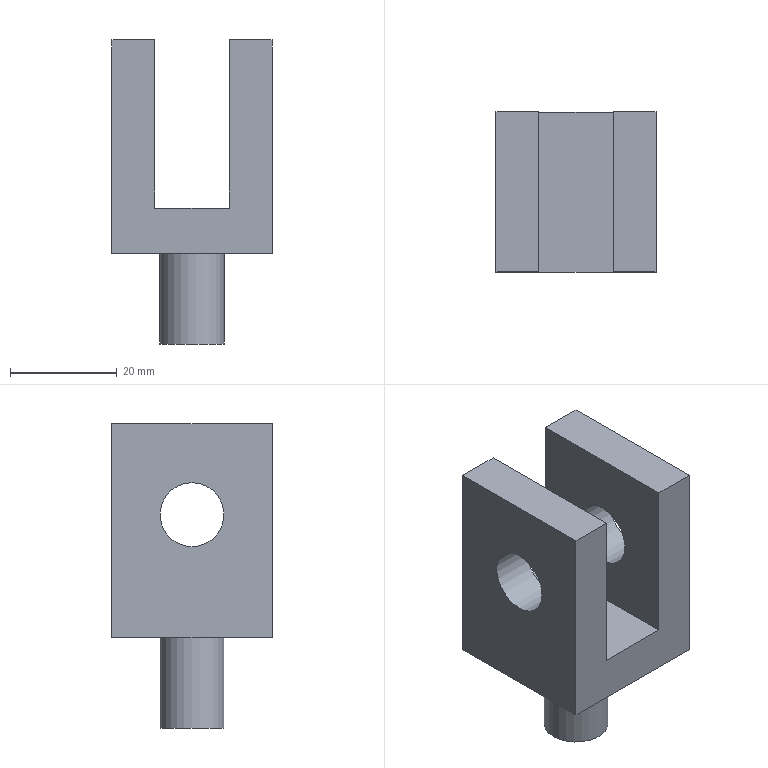Component | NX | HINGE_LINK | 1 solid | 14 faces | box 30 x 30 x 57 mm | volume 22883 mm3 | plane 11 | cylinder 3 | commonest cylinder face diameters 12 x3
STEP:
#1=CARTESIAN_POINT('',(0.,0.,0.));
#2=DIRECTION('',(0.,0.,1.));
#3=DIRECTION('',(1.,0.,0.));
#4=AXIS2_PLACEMENT_3D('',#1,#2,#3);
#5=CARTESIAN_POINT('',(545.625,-110.909,-15.057));
#6=VERTEX_POINT('',#5);
#7=CARTESIAN_POINT('',(553.625,-110.909,-15.057));
#8=VERTEX_POINT('',#7);
#9=CARTESIAN_POINT('',(545.625,-110.909,-15.057));
#10=DIRECTION('',(1.,0.,0.));
#11=VECTOR('',#10,1.);
#12=LINE('',#9,#11);
#13=CARTESIAN_POINT('',(560.625,-95.909,-15.057));
#14=DIRECTION('',(0.,0.,1.));
#15=DIRECTION('',(1.,0.,0.));
#16=AXIS2_PLACEMENT_3D('',#13,#14,#15);
#17=PLANE('',#16);
#18=CARTESIAN_POINT('',(-15.,-15.));
#19=DIRECTION('',(1.,0.));
#20=VECTOR('',#19,1.);
#21=LINE('',#18,#20);
#22=(GEOMETRIC_REPRESENTATION_CONTEXT(2)PARAMETRIC_REPRESENTATION_CONTEXT()REPRESENTATION_CONTEXT('',''));
#23=DEFINITIONAL_REPRESENTATION('',(#21),#22);
#24=PCURVE('',#17,#23);
#25=CARTESIAN_POINT('',(545.625,-110.909,-10.057));
#26=DIRECTION('',(0.,1.,0.));
#27=DIRECTION('',(0.,0.,1.));
#28=AXIS2_PLACEMENT_3D('',#25,#26,#27);
#29=PLANE('',#28);
#30=CARTESIAN_POINT('',(-5.,0.));
#31=DIRECTION('',(0.,1.));
#32=VECTOR('',#31,1.);
#33=LINE('',#30,#32);
#34=(GEOMETRIC_REPRESENTATION_CONTEXT(2)PARAMETRIC_REPRESENTATION_CONTEXT()REPRESENTATION_CONTEXT('',''));
#35=DEFINITIONAL_REPRESENTATION('',(#33),#34);
#36=PCURVE('',#29,#35);
#37=SURFACE_CURVE('',#12,(#24,#36),.PCURVE_S1.);
#38=EDGE_CURVE('',#6,#8,#37,.T.);
#39=ORIENTED_EDGE('',*,*,#38,.T.);
#40=CARTESIAN_POINT('',(553.625,-80.909,-15.057));
#41=VERTEX_POINT('',#40);
#42=CARTESIAN_POINT('',(553.625,-95.909,-15.057));
#43=DIRECTION('',(0.,1.,0.));
#44=VECTOR('',#43,1.);
#45=LINE('',#42,#44);
#46=CARTESIAN_POINT('',(-7.,0.));
#47=DIRECTION('',(0.,1.));
#48=VECTOR('',#47,1.);
#49=LINE('',#46,#48);
#50=(GEOMETRIC_REPRESENTATION_CONTEXT(2)PARAMETRIC_REPRESENTATION_CONTEXT()REPRESENTATION_CONTEXT('',''));
#51=DEFINITIONAL_REPRESENTATION('',(#49),#50);
#52=PCURVE('',#17,#51);
#53=CARTESIAN_POINT('',(553.625,-95.909,-72.057));
#54=DIRECTION('',(1.,0.,0.));
#55=DIRECTION('',(0.,0.,-1.));
#56=AXIS2_PLACEMENT_3D('',#53,#54,#55);
#57=PLANE('',#56);
#58=CARTESIAN_POINT('',(-57.,0.));
#59=DIRECTION('',(0.,1.));
#60=VECTOR('',#59,1.);
#61=LINE('',#58,#60);
#62=(GEOMETRIC_REPRESENTATION_CONTEXT(2)PARAMETRIC_REPRESENTATION_CONTEXT()REPRESENTATION_CONTEXT('',''));
#63=DEFINITIONAL_REPRESENTATION('',(#61),#62);
#64=PCURVE('',#57,#63);
#65=SURFACE_CURVE('',#45,(#52,#64),.PCURVE_S1.);
#66=EDGE_CURVE('',#8,#41,#65,.T.);
#67=ORIENTED_EDGE('',*,*,#66,.T.);
#68=CARTESIAN_POINT('',(545.625,-80.909,-15.057));
#69=VERTEX_POINT('',#68);
#70=CARTESIAN_POINT('',(575.625,-80.909,-15.057));
#71=DIRECTION('',(-1.,0.,0.));
#72=VECTOR('',#71,1.);
#73=LINE('',#70,#72);
#74=CARTESIAN_POINT('',(15.,15.));
#75=DIRECTION('',(-1.,0.));
#76=VECTOR('',#75,1.);
#77=LINE('',#74,#76);
#78=(GEOMETRIC_REPRESENTATION_CONTEXT(2)PARAMETRIC_REPRESENTATION_CONTEXT()REPRESENTATION_CONTEXT('',''));
#79=DEFINITIONAL_REPRESENTATION('',(#77),#78);
#80=PCURVE('',#17,#79);
#81=CARTESIAN_POINT('',(575.625,-80.909,-10.057));
#82=DIRECTION('',(0.,-1.,0.));
#83=DIRECTION('',(0.,0.,-1.));
#84=AXIS2_PLACEMENT_3D('',#81,#82,#83);
#85=PLANE('',#84);
#86=CARTESIAN_POINT('',(5.,0.));
#87=DIRECTION('',(0.,-1.));
#88=VECTOR('',#87,1.);
#89=LINE('',#86,#88);
#90=(GEOMETRIC_REPRESENTATION_CONTEXT(2)PARAMETRIC_REPRESENTATION_CONTEXT()REPRESENTATION_CONTEXT('',''));
#91=DEFINITIONAL_REPRESENTATION('',(#89),#90);
#92=PCURVE('',#85,#91);
#93=SURFACE_CURVE('',#73,(#80,#92),.PCURVE_S1.);
#94=EDGE_CURVE('',#41,#69,#93,.T.);
#95=ORIENTED_EDGE('',*,*,#94,.T.);
#96=CARTESIAN_POINT('',(545.625,-80.909,-15.057));
#97=DIRECTION('',(0.,-1.,0.));
#98=VECTOR('',#97,1.);
#99=LINE('',#96,#98);
#100=CARTESIAN_POINT('',(-15.,15.));
#101=DIRECTION('',(0.,-1.));
#102=VECTOR('',#101,1.);
#103=LINE('',#100,#102);
#104=(GEOMETRIC_REPRESENTATION_CONTEXT(2)PARAMETRIC_REPRESENTATION_CONTEXT()REPRESENTATION_CONTEXT('',''));
#105=DEFINITIONAL_REPRESENTATION('',(#103),#104);
#106=PCURVE('',#17,#105);
#107=CARTESIAN_POINT('',(545.625,-80.909,-10.057));
#108=DIRECTION('',(1.,0.,0.));
#109=DIRECTION('',(0.,0.,-1.));
#110=AXIS2_PLACEMENT_3D('',#107,#108,#109);
#111=PLANE('',#110);
#112=CARTESIAN_POINT('',(5.,0.));
#113=DIRECTION('',(0.,-1.));
#114=VECTOR('',#113,1.);
#115=LINE('',#112,#114);
#116=(GEOMETRIC_REPRESENTATION_CONTEXT(2)PARAMETRIC_REPRESENTATION_CONTEXT()REPRESENTATION_CONTEXT('',''));
#117=DEFINITIONAL_REPRESENTATION('',(#115),#116);
#118=PCURVE('',#111,#117);
#119=SURFACE_CURVE('',#99,(#106,#118),.PCURVE_S1.);
#120=EDGE_CURVE('',#69,#6,#119,.T.);
#121=ORIENTED_EDGE('',*,*,#120,.T.);
#122=EDGE_LOOP('',(#39,#67,#95,#121));
#123=FACE_BOUND('',#122,.T.);
#124=ADVANCED_FACE('',(#123),#17,.T.);
#125=CARTESIAN_POINT('',(566.625,-95.909,-72.057));
#126=VERTEX_POINT('',#125);
#127=CARTESIAN_POINT('',(560.625,-95.909,-72.057));
#128=DIRECTION('',(0.,0.,1.));
#129=DIRECTION('',(1.,0.,0.));
#130=AXIS2_PLACEMENT_3D('',#127,#128,#129);
#131=CIRCLE('',#130,6.);
#132=CARTESIAN_POINT('',(560.625,-95.909,-72.057));
#133=DIRECTION('',(0.,0.,-1.));
#134=DIRECTION('',(-1.,0.,0.));
#135=AXIS2_PLACEMENT_3D('',#132,#133,#134);
#136=PLANE('',#135);
#137=CARTESIAN_POINT('',(-6.,0.));
#138=CARTESIAN_POINT('',(-6.,10.392));
#139=CARTESIAN_POINT('',(3.,5.196));
#140=CARTESIAN_POINT('',(12.,0.));
#141=CARTESIAN_POINT('',(3.,-5.196));
#142=CARTESIAN_POINT('',(-6.,-10.392));
#143=CARTESIAN_POINT('',(-6.,0.));
#144=(BOUNDED_CURVE()B_SPLINE_CURVE(2,(#137,#138,#139,#140,#141,#142,#143),.UNSPECIFIED.,.T.,.F.)B_SPLINE_CURVE_WITH_KNOTS((1,2,2,2,2,1),(-2.094,0.,2.094,4.189,6.283,8.378),.UNSPECIFIED.)CURVE()GEOMETRIC_REPRESENTATION_ITEM()RATIONAL_B_SPLINE_CURVE((1.,0.5,1.,0.5,1.,0.5,1.))REPRESENTATION_ITEM(''));
#145=(GEOMETRIC_REPRESENTATION_CONTEXT(2)PARAMETRIC_REPRESENTATION_CONTEXT()REPRESENTATION_CONTEXT('',''));
#146=DEFINITIONAL_REPRESENTATION('',(#144),#145);
#147=PCURVE('',#136,#146);
#148=CARTESIAN_POINT('',(560.625,-95.909,-72.057));
#149=DIRECTION('',(0.,0.,1.));
#150=DIRECTION('',(1.,0.,0.));
#151=AXIS2_PLACEMENT_3D('',#148,#149,#150);
#152=CYLINDRICAL_SURFACE('',#151,6.);
#153=CARTESIAN_POINT('',(0.,0.));
#154=DIRECTION('',(1.,0.));
#155=VECTOR('',#154,1.);
#156=LINE('',#153,#155);
#157=(GEOMETRIC_REPRESENTATION_CONTEXT(2)PARAMETRIC_REPRESENTATION_CONTEXT()REPRESENTATION_CONTEXT('',''));
#158=DEFINITIONAL_REPRESENTATION('',(#156),#157);
#159=PCURVE('',#152,#158);
#160=SURFACE_CURVE('',#131,(#147,#159),.PCURVE_S1.);
#161=EDGE_CURVE('',#126,#126,#160,.T.);
#162=ORIENTED_EDGE('',*,*,#161,.F.);
#163=EDGE_LOOP('',(#162));
#164=FACE_BOUND('',#163,.T.);
#165=ADVANCED_FACE('',(#164),#136,.T.);
#166=CARTESIAN_POINT('',(566.625,-95.909,-55.057));
#167=VERTEX_POINT('',#166);
#168=CARTESIAN_POINT('',(560.625,-95.909,-55.057));
#169=DIRECTION('',(0.,0.,-1.));
#170=DIRECTION('',(1.,0.,0.));
#171=AXIS2_PLACEMENT_3D('',#168,#169,#170);
#172=CIRCLE('',#171,6.);
#173=CARTESIAN_POINT('',(6.283,17.));
#174=DIRECTION('',(-1.,0.));
#175=VECTOR('',#174,1.);
#176=LINE('',#173,#175);
#177=(GEOMETRIC_REPRESENTATION_CONTEXT(2)PARAMETRIC_REPRESENTATION_CONTEXT()REPRESENTATION_CONTEXT('',''));
#178=DEFINITIONAL_REPRESENTATION('',(#176),#177);
#179=PCURVE('',#152,#178);
#180=CARTESIAN_POINT('',(560.625,-95.909,-55.057));
#181=DIRECTION('',(0.,0.,1.));
#182=DIRECTION('',(1.,0.,0.));
#183=AXIS2_PLACEMENT_3D('',#180,#181,#182);
#184=PLANE('',#183);
#185=CARTESIAN_POINT('',(6.,0.));
#186=CARTESIAN_POINT('',(6.,-10.392));
#187=CARTESIAN_POINT('',(-3.,-5.196));
#188=CARTESIAN_POINT('',(-12.,-0.));
#189=CARTESIAN_POINT('',(-3.,5.196));
#190=CARTESIAN_POINT('',(6.,10.392));
#191=CARTESIAN_POINT('',(6.,0.));
#192=(BOUNDED_CURVE()B_SPLINE_CURVE(2,(#185,#186,#187,#188,#189,#190,#191),.UNSPECIFIED.,.T.,.F.)B_SPLINE_CURVE_WITH_KNOTS((1,2,2,2,2,1),(-2.094,0.,2.094,4.189,6.283,8.378),.UNSPECIFIED.)CURVE()GEOMETRIC_REPRESENTATION_ITEM()RATIONAL_B_SPLINE_CURVE((1.,0.5,1.,0.5,1.,0.5,1.))REPRESENTATION_ITEM(''));
#193=(GEOMETRIC_REPRESENTATION_CONTEXT(2)PARAMETRIC_REPRESENTATION_CONTEXT()REPRESENTATION_CONTEXT('',''));
#194=DEFINITIONAL_REPRESENTATION('',(#192),#193);
#195=PCURVE('',#184,#194);
#196=SURFACE_CURVE('',#172,(#179,#195),.PCURVE_S1.);
#197=EDGE_CURVE('',#167,#167,#196,.T.);
#198=ORIENTED_EDGE('',*,*,#197,.T.);
#199=CARTESIAN_POINT('',(566.625,-95.909,-72.057));
#200=CARTESIAN_POINT('',(566.625,-95.909,-55.057));
#201=B_SPLINE_CURVE_WITH_KNOTS('',1,(#199,#200),.UNSPECIFIED.,.F.,.F.,(2,2),(0.,17.),.PIECEWISE_BEZIER_KNOTS.);
#202=CARTESIAN_POINT('',(0.,0.));
#203=DIRECTION('',(0.,1.));
#204=VECTOR('',#203,1.);
#205=LINE('',#202,#204);
#206=(GEOMETRIC_REPRESENTATION_CONTEXT(2)PARAMETRIC_REPRESENTATION_CONTEXT()REPRESENTATION_CONTEXT('',''));
#207=DEFINITIONAL_REPRESENTATION('',(#205),#206);
#208=PCURVE('',#152,#207);
#209=CARTESIAN_POINT('',(6.283,0.));
#210=DIRECTION('',(0.,1.));
#211=VECTOR('',#210,1.);
#212=LINE('',#209,#211);
#213=(GEOMETRIC_REPRESENTATION_CONTEXT(2)PARAMETRIC_REPRESENTATION_CONTEXT()REPRESENTATION_CONTEXT('',''));
#214=DEFINITIONAL_REPRESENTATION('',(#212),#213);
#215=PCURVE('',#152,#214);
#216=SEAM_CURVE('',#201,(#208,#215),.PCURVE_S1.);
#217=EDGE_CURVE('',#126,#167,#216,.T.);
#218=ORIENTED_EDGE('',*,*,#217,.F.);
#219=ORIENTED_EDGE('',*,*,#161,.T.);
#220=ORIENTED_EDGE('',*,*,#217,.T.);
#221=EDGE_LOOP('',(#198,#218,#219,#220));
#222=FACE_BOUND('',#221,.T.);
#223=ADVANCED_FACE('',(#222),#152,.T.);
#224=CARTESIAN_POINT('',(545.625,-95.909,-38.057));
#225=VERTEX_POINT('',#224);
#226=CARTESIAN_POINT('',(545.625,-95.909,-32.057));
#227=DIRECTION('',(-1.,0.,0.));
#228=DIRECTION('',(0.,0.,-1.));
#229=AXIS2_PLACEMENT_3D('',#226,#227,#228);
#230=CIRCLE('',#229,6.);
#231=CARTESIAN_POINT('',(28.,-15.));
#232=CARTESIAN_POINT('',(28.,-25.392));
#233=CARTESIAN_POINT('',(19.,-20.196));
#234=CARTESIAN_POINT('',(10.,-15.));
#235=CARTESIAN_POINT('',(19.,-9.804));
#236=CARTESIAN_POINT('',(28.,-4.608));
#237=CARTESIAN_POINT('',(28.,-15.));
#238=(BOUNDED_CURVE()B_SPLINE_CURVE(2,(#231,#232,#233,#234,#235,#236,#237),.UNSPECIFIED.,.T.,.F.)B_SPLINE_CURVE_WITH_KNOTS((1,2,2,2,2,1),(-2.094,0.,2.094,4.189,6.283,8.378),.UNSPECIFIED.)CURVE()GEOMETRIC_REPRESENTATION_ITEM()RATIONAL_B_SPLINE_CURVE((1.,0.5,1.,0.5,1.,0.5,1.))REPRESENTATION_ITEM(''));
#239=(GEOMETRIC_REPRESENTATION_CONTEXT(2)PARAMETRIC_REPRESENTATION_CONTEXT()REPRESENTATION_CONTEXT('',''));
#240=DEFINITIONAL_REPRESENTATION('',(#238),#239);
#241=PCURVE('',#111,#240);
#242=CARTESIAN_POINT('',(591.625,-95.909,-32.057));
#243=DIRECTION('',(-1.,0.,0.));
#244=DIRECTION('',(0.,0.,1.));
#245=AXIS2_PLACEMENT_3D('',#242,#243,#244);
#246=CYLINDRICAL_SURFACE('',#245,6.);
#247=CARTESIAN_POINT('',(3.142,46.));
#248=DIRECTION('',(1.,0.));
#249=VECTOR('',#248,1.);
#250=LINE('',#247,#249);
#251=(GEOMETRIC_REPRESENTATION_CONTEXT(2)PARAMETRIC_REPRESENTATION_CONTEXT()REPRESENTATION_CONTEXT('',''));
#252=DEFINITIONAL_REPRESENTATION('',(#250),#251);
#253=PCURVE('',#246,#252);
#254=SURFACE_CURVE('',#230,(#241,#253),.PCURVE_S1.);
#255=EDGE_CURVE('',#225,#225,#254,.T.);
#256=ORIENTED_EDGE('',*,*,#255,.F.);
#257=EDGE_LOOP('',(#256));
#258=FACE_BOUND('',#257,.T.);
#259=CARTESIAN_POINT('',(545.625,-80.909,-55.057));
#260=VERTEX_POINT('',#259);
#261=CARTESIAN_POINT('',(545.625,-110.909,-55.057));
#262=VERTEX_POINT('',#261);
#263=CARTESIAN_POINT('',(545.625,-80.909,-55.057));
#264=DIRECTION('',(0.,-1.,0.));
#265=VECTOR('',#264,1.);
#266=LINE('',#263,#265);
#267=CARTESIAN_POINT('',(45.,0.));
#268=DIRECTION('',(0.,-1.));
#269=VECTOR('',#268,1.);
#270=LINE('',#267,#269);
#271=(GEOMETRIC_REPRESENTATION_CONTEXT(2)PARAMETRIC_REPRESENTATION_CONTEXT()REPRESENTATION_CONTEXT('',''));
#272=DEFINITIONAL_REPRESENTATION('',(#270),#271);
#273=PCURVE('',#111,#272);
#274=CARTESIAN_POINT('',(-15.,15.));
#275=DIRECTION('',(0.,-1.));
#276=VECTOR('',#275,1.);
#277=LINE('',#274,#276);
#278=(GEOMETRIC_REPRESENTATION_CONTEXT(2)PARAMETRIC_REPRESENTATION_CONTEXT()REPRESENTATION_CONTEXT('',''));
#279=DEFINITIONAL_REPRESENTATION('',(#277),#278);
#280=PCURVE('',#184,#279);
#281=SURFACE_CURVE('',#266,(#273,#280),.PCURVE_S1.);
#282=EDGE_CURVE('',#260,#262,#281,.T.);
#283=ORIENTED_EDGE('',*,*,#282,.T.);
#284=CARTESIAN_POINT('',(545.625,-110.909,-10.057));
#285=DIRECTION('',(0.,0.,-1.));
#286=VECTOR('',#285,1.);
#287=LINE('',#284,#286);
#288=CARTESIAN_POINT('',(0.,-30.));
#289=DIRECTION('',(1.,0.));
#290=VECTOR('',#289,1.);
#291=LINE('',#288,#290);
#292=(GEOMETRIC_REPRESENTATION_CONTEXT(2)PARAMETRIC_REPRESENTATION_CONTEXT()REPRESENTATION_CONTEXT('',''));
#293=DEFINITIONAL_REPRESENTATION('',(#291),#292);
#294=PCURVE('',#111,#293);
#295=CARTESIAN_POINT('',(0.,0.));
#296=DIRECTION('',(-1.,0.));
#297=VECTOR('',#296,1.);
#298=LINE('',#295,#297);
#299=(GEOMETRIC_REPRESENTATION_CONTEXT(2)PARAMETRIC_REPRESENTATION_CONTEXT()REPRESENTATION_CONTEXT('',''));
#300=DEFINITIONAL_REPRESENTATION('',(#298),#299);
#301=PCURVE('',#29,#300);
#302=SURFACE_CURVE('',#287,(#294,#301),.PCURVE_S1.);
#303=EDGE_CURVE('',#6,#262,#302,.T.);
#304=ORIENTED_EDGE('',*,*,#303,.F.);
#305=ORIENTED_EDGE('',*,*,#120,.F.);
#306=CARTESIAN_POINT('',(545.625,-80.909,-10.057));
#307=DIRECTION('',(0.,0.,-1.));
#308=VECTOR('',#307,1.);
#309=LINE('',#306,#308);
#310=CARTESIAN_POINT('',(0.,0.));
#311=DIRECTION('',(1.,0.));
#312=VECTOR('',#311,1.);
#313=LINE('',#310,#312);
#314=(GEOMETRIC_REPRESENTATION_CONTEXT(2)PARAMETRIC_REPRESENTATION_CONTEXT()REPRESENTATION_CONTEXT('',''));
#315=DEFINITIONAL_REPRESENTATION('',(#313),#314);
#316=PCURVE('',#111,#315);
#317=CARTESIAN_POINT('',(0.,-30.));
#318=DIRECTION('',(1.,0.));
#319=VECTOR('',#318,1.);
#320=LINE('',#317,#319);
#321=(GEOMETRIC_REPRESENTATION_CONTEXT(2)PARAMETRIC_REPRESENTATION_CONTEXT()REPRESENTATION_CONTEXT('',''));
#322=DEFINITIONAL_REPRESENTATION('',(#320),#321);
#323=PCURVE('',#85,#322);
#324=SURFACE_CURVE('',#309,(#316,#323),.PCURVE_S1.);
#325=EDGE_CURVE('',#69,#260,#324,.T.);
#326=ORIENTED_EDGE('',*,*,#325,.T.);
#327=EDGE_LOOP('',(#283,#304,#305,#326));
#328=FACE_BOUND('',#327,.T.);
#329=ADVANCED_FACE('',(#258,#328),#111,.F.);
#330=CARTESIAN_POINT('',(567.625,-110.909,-15.057));
#331=VERTEX_POINT('',#330);
#332=CARTESIAN_POINT('',(575.625,-110.909,-15.057));
#333=VERTEX_POINT('',#332);
#334=CARTESIAN_POINT('',(545.625,-110.909,-15.057));
#335=DIRECTION('',(1.,0.,0.));
#336=VECTOR('',#335,1.);
#337=LINE('',#334,#336);
#338=CARTESIAN_POINT('',(-5.,0.));
#339=DIRECTION('',(0.,1.));
#340=VECTOR('',#339,1.);
#341=LINE('',#338,#340);
#342=(GEOMETRIC_REPRESENTATION_CONTEXT(2)PARAMETRIC_REPRESENTATION_CONTEXT()REPRESENTATION_CONTEXT('',''));
#343=DEFINITIONAL_REPRESENTATION('',(#341),#342);
#344=PCURVE('',#29,#343);
#345=CARTESIAN_POINT('',(560.625,-95.909,-15.057));
#346=DIRECTION('',(0.,0.,1.));
#347=DIRECTION('',(1.,0.,0.));
#348=AXIS2_PLACEMENT_3D('',#345,#346,#347);
#349=PLANE('',#348);
#350=CARTESIAN_POINT('',(-15.,-15.));
#351=DIRECTION('',(1.,0.));
#352=VECTOR('',#351,1.);
#353=LINE('',#350,#352);
#354=(GEOMETRIC_REPRESENTATION_CONTEXT(2)PARAMETRIC_REPRESENTATION_CONTEXT()REPRESENTATION_CONTEXT('',''));
#355=DEFINITIONAL_REPRESENTATION('',(#353),#354);
#356=PCURVE('',#349,#355);
#357=SURFACE_CURVE('',#337,(#344,#356),.PCURVE_S1.);
#358=EDGE_CURVE('',#331,#333,#357,.T.);
#359=ORIENTED_EDGE('',*,*,#358,.F.);
#360=CARTESIAN_POINT('',(567.625,-110.909,-46.557));
#361=VERTEX_POINT('',#360);
#362=CARTESIAN_POINT('',(567.625,-110.909,-10.057));
#363=DIRECTION('',(0.,0.,-1.));
#364=VECTOR('',#363,1.);
#365=LINE('',#362,#364);
#366=CARTESIAN_POINT('',(0.,22.));
#367=DIRECTION('',(-1.,0.));
#368=VECTOR('',#367,1.);
#369=LINE('',#366,#368);
#370=(GEOMETRIC_REPRESENTATION_CONTEXT(2)PARAMETRIC_REPRESENTATION_CONTEXT()REPRESENTATION_CONTEXT('',''));
#371=DEFINITIONAL_REPRESENTATION('',(#369),#370);
#372=PCURVE('',#29,#371);
#373=CARTESIAN_POINT('',(567.625,-95.909,-72.057));
#374=DIRECTION('',(1.,0.,0.));
#375=DIRECTION('',(0.,0.,-1.));
#376=AXIS2_PLACEMENT_3D('',#373,#374,#375);
#377=PLANE('',#376);
#378=CARTESIAN_POINT('',(-62.,-15.));
#379=DIRECTION('',(1.,0.));
#380=VECTOR('',#379,1.);
#381=LINE('',#378,#380);
#382=(GEOMETRIC_REPRESENTATION_CONTEXT(2)PARAMETRIC_REPRESENTATION_CONTEXT()REPRESENTATION_CONTEXT('',''));
#383=DEFINITIONAL_REPRESENTATION('',(#381),#382);
#384=PCURVE('',#377,#383);
#385=SURFACE_CURVE('',#365,(#372,#384),.PCURVE_S1.);
#386=EDGE_CURVE('',#331,#361,#385,.T.);
#387=ORIENTED_EDGE('',*,*,#386,.T.);
#388=CARTESIAN_POINT('',(553.625,-110.909,-46.557));
#389=VERTEX_POINT('',#388);
#390=CARTESIAN_POINT('',(545.625,-110.909,-46.557));
#391=DIRECTION('',(1.,0.,0.));
#392=VECTOR('',#391,1.);
#393=LINE('',#390,#392);
#394=CARTESIAN_POINT('',(-36.5,0.));
#395=DIRECTION('',(0.,1.));
#396=VECTOR('',#395,1.);
#397=LINE('',#394,#396);
#398=(GEOMETRIC_REPRESENTATION_CONTEXT(2)PARAMETRIC_REPRESENTATION_CONTEXT()REPRESENTATION_CONTEXT('',''));
#399=DEFINITIONAL_REPRESENTATION('',(#397),#398);
#400=PCURVE('',#29,#399);
#401=CARTESIAN_POINT('',(567.625,-135.909,-46.557));
#402=DIRECTION('',(0.,-0.,1.));
#403=DIRECTION('',(0.,-1.,-0.));
#404=AXIS2_PLACEMENT_3D('',#401,#402,#403);
#405=PLANE('',#404);
#406=CARTESIAN_POINT('',(-25.,-22.));
#407=DIRECTION('',(0.,1.));
#408=VECTOR('',#407,1.);
#409=LINE('',#406,#408);
#410=(GEOMETRIC_REPRESENTATION_CONTEXT(2)PARAMETRIC_REPRESENTATION_CONTEXT()REPRESENTATION_CONTEXT('',''));
#411=DEFINITIONAL_REPRESENTATION('',(#409),#410);
#412=PCURVE('',#405,#411);
#413=SURFACE_CURVE('',#393,(#400,#412),.PCURVE_S1.);
#414=EDGE_CURVE('',#389,#361,#413,.T.);
#415=ORIENTED_EDGE('',*,*,#414,.F.);
#416=CARTESIAN_POINT('',(553.625,-110.909,-10.057));
#417=DIRECTION('',(0.,0.,-1.));
#418=VECTOR('',#417,1.);
#419=LINE('',#416,#418);
#420=CARTESIAN_POINT('',(0.,8.));
#421=DIRECTION('',(-1.,0.));
#422=VECTOR('',#421,1.);
#423=LINE('',#420,#422);
#424=(GEOMETRIC_REPRESENTATION_CONTEXT(2)PARAMETRIC_REPRESENTATION_CONTEXT()REPRESENTATION_CONTEXT('',''));
#425=DEFINITIONAL_REPRESENTATION('',(#423),#424);
#426=PCURVE('',#29,#425);
#427=CARTESIAN_POINT('',(-62.,-15.));
#428=DIRECTION('',(1.,0.));
#429=VECTOR('',#428,1.);
#430=LINE('',#427,#429);
#431=(GEOMETRIC_REPRESENTATION_CONTEXT(2)PARAMETRIC_REPRESENTATION_CONTEXT()REPRESENTATION_CONTEXT('',''));
#432=DEFINITIONAL_REPRESENTATION('',(#430),#431);
#433=PCURVE('',#57,#432);
#434=SURFACE_CURVE('',#419,(#426,#433),.PCURVE_S1.);
#435=EDGE_CURVE('',#8,#389,#434,.T.);
#436=ORIENTED_EDGE('',*,*,#435,.F.);
#437=ORIENTED_EDGE('',*,*,#38,.F.);
#438=ORIENTED_EDGE('',*,*,#303,.T.);
#439=CARTESIAN_POINT('',(575.625,-110.909,-55.057));
#440=VERTEX_POINT('',#439);
#441=CARTESIAN_POINT('',(545.625,-110.909,-55.057));
#442=DIRECTION('',(1.,0.,0.));
#443=VECTOR('',#442,1.);
#444=LINE('',#441,#443);
#445=CARTESIAN_POINT('',(-45.,0.));
#446=DIRECTION('',(0.,1.));
#447=VECTOR('',#446,1.);
#448=LINE('',#445,#447);
#449=(GEOMETRIC_REPRESENTATION_CONTEXT(2)PARAMETRIC_REPRESENTATION_CONTEXT()REPRESENTATION_CONTEXT('',''));
#450=DEFINITIONAL_REPRESENTATION('',(#448),#449);
#451=PCURVE('',#29,#450);
#452=CARTESIAN_POINT('',(-15.,-15.));
#453=DIRECTION('',(1.,0.));
#454=VECTOR('',#453,1.);
#455=LINE('',#452,#454);
#456=(GEOMETRIC_REPRESENTATION_CONTEXT(2)PARAMETRIC_REPRESENTATION_CONTEXT()REPRESENTATION_CONTEXT('',''));
#457=DEFINITIONAL_REPRESENTATION('',(#455),#456);
#458=PCURVE('',#184,#457);
#459=SURFACE_CURVE('',#444,(#451,#458),.PCURVE_S1.);
#460=EDGE_CURVE('',#262,#440,#459,.T.);
#461=ORIENTED_EDGE('',*,*,#460,.T.);
#462=CARTESIAN_POINT('',(575.625,-110.909,-10.057));
#463=DIRECTION('',(0.,0.,-1.));
#464=VECTOR('',#463,1.);
#465=LINE('',#462,#464);
#466=CARTESIAN_POINT('',(0.,30.));
#467=DIRECTION('',(-1.,0.));
#468=VECTOR('',#467,1.);
#469=LINE('',#466,#468);
#470=(GEOMETRIC_REPRESENTATION_CONTEXT(2)PARAMETRIC_REPRESENTATION_CONTEXT()REPRESENTATION_CONTEXT('',''));
#471=DEFINITIONAL_REPRESENTATION('',(#469),#470);
#472=PCURVE('',#29,#471);
#473=CARTESIAN_POINT('',(575.625,-110.909,-10.057));
#474=DIRECTION('',(-1.,0.,0.));
#475=DIRECTION('',(0.,0.,1.));
#476=AXIS2_PLACEMENT_3D('',#473,#474,#475);
#477=PLANE('',#476);
#478=CARTESIAN_POINT('',(0.,0.));
#479=DIRECTION('',(-1.,0.));
#480=VECTOR('',#479,1.);
#481=LINE('',#478,#480);
#482=(GEOMETRIC_REPRESENTATION_CONTEXT(2)PARAMETRIC_REPRESENTATION_CONTEXT()REPRESENTATION_CONTEXT('',''));
#483=DEFINITIONAL_REPRESENTATION('',(#481),#482);
#484=PCURVE('',#477,#483);
#485=SURFACE_CURVE('',#465,(#472,#484),.PCURVE_S1.);
#486=EDGE_CURVE('',#333,#440,#485,.T.);
#487=ORIENTED_EDGE('',*,*,#486,.F.);
#488=EDGE_LOOP('',(#359,#387,#415,#436,#437,#438,#461,#487));
#489=FACE_BOUND('',#488,.T.);
#490=ADVANCED_FACE('',(#489),#29,.F.);
#491=CARTESIAN_POINT('',(575.625,-95.909,-26.057));
#492=VERTEX_POINT('',#491);
#493=CARTESIAN_POINT('',(575.625,-95.909,-32.057));
#494=DIRECTION('',(1.,0.,0.));
#495=DIRECTION('',(0.,0.,1.));
#496=AXIS2_PLACEMENT_3D('',#493,#494,#495);
#497=CIRCLE('',#496,6.);
#498=CARTESIAN_POINT('',(-16.,15.));
#499=CARTESIAN_POINT('',(-16.,4.608));
#500=CARTESIAN_POINT('',(-25.,9.804));
#501=CARTESIAN_POINT('',(-34.,15.));
#502=CARTESIAN_POINT('',(-25.,20.196));
#503=CARTESIAN_POINT('',(-16.,25.392));
#504=CARTESIAN_POINT('',(-16.,15.));
#505=(BOUNDED_CURVE()B_SPLINE_CURVE(2,(#498,#499,#500,#501,#502,#503,#504),.UNSPECIFIED.,.T.,.F.)B_SPLINE_CURVE_WITH_KNOTS((1,2,2,2,2,1),(-2.094,0.,2.094,4.189,6.283,8.378),.UNSPECIFIED.)CURVE()GEOMETRIC_REPRESENTATION_ITEM()RATIONAL_B_SPLINE_CURVE((1.,0.5,1.,0.5,1.,0.5,1.))REPRESENTATION_ITEM(''));
#506=(GEOMETRIC_REPRESENTATION_CONTEXT(2)PARAMETRIC_REPRESENTATION_CONTEXT()REPRESENTATION_CONTEXT('',''));
#507=DEFINITIONAL_REPRESENTATION('',(#505),#506);
#508=PCURVE('',#477,#507);
#509=CARTESIAN_POINT('',(591.625,-95.909,-32.057));
#510=DIRECTION('',(-1.,0.,0.));
#511=DIRECTION('',(0.,0.,1.));
#512=AXIS2_PLACEMENT_3D('',#509,#510,#511);
#513=CYLINDRICAL_SURFACE('',#512,6.);
#514=CARTESIAN_POINT('',(6.283,16.));
#515=DIRECTION('',(-1.,0.));
#516=VECTOR('',#515,1.);
#517=LINE('',#514,#516);
#518=(GEOMETRIC_REPRESENTATION_CONTEXT(2)PARAMETRIC_REPRESENTATION_CONTEXT()REPRESENTATION_CONTEXT('',''));
#519=DEFINITIONAL_REPRESENTATION('',(#517),#518);
#520=PCURVE('',#513,#519);
#521=SURFACE_CURVE('',#497,(#508,#520),.PCURVE_S1.);
#522=EDGE_CURVE('',#492,#492,#521,.T.);
#523=ORIENTED_EDGE('',*,*,#522,.F.);
#524=EDGE_LOOP('',(#523));
#525=FACE_BOUND('',#524,.T.);
#526=CARTESIAN_POINT('',(575.625,-80.909,-55.057));
#527=VERTEX_POINT('',#526);
#528=CARTESIAN_POINT('',(575.625,-110.909,-55.057));
#529=DIRECTION('',(0.,1.,0.));
#530=VECTOR('',#529,1.);
#531=LINE('',#528,#530);
#532=CARTESIAN_POINT('',(-45.,0.));
#533=DIRECTION('',(0.,1.));
#534=VECTOR('',#533,1.);
#535=LINE('',#532,#534);
#536=(GEOMETRIC_REPRESENTATION_CONTEXT(2)PARAMETRIC_REPRESENTATION_CONTEXT()REPRESENTATION_CONTEXT('',''));
#537=DEFINITIONAL_REPRESENTATION('',(#535),#536);
#538=PCURVE('',#477,#537);
#539=CARTESIAN_POINT('',(15.,-15.));
#540=DIRECTION('',(0.,1.));
#541=VECTOR('',#540,1.);
#542=LINE('',#539,#541);
#543=(GEOMETRIC_REPRESENTATION_CONTEXT(2)PARAMETRIC_REPRESENTATION_CONTEXT()REPRESENTATION_CONTEXT('',''));
#544=DEFINITIONAL_REPRESENTATION('',(#542),#543);
#545=PCURVE('',#184,#544);
#546=SURFACE_CURVE('',#531,(#538,#545),.PCURVE_S1.);
#547=EDGE_CURVE('',#440,#527,#546,.T.);
#548=ORIENTED_EDGE('',*,*,#547,.T.);
#549=CARTESIAN_POINT('',(575.625,-80.909,-15.057));
#550=VERTEX_POINT('',#549);
#551=CARTESIAN_POINT('',(575.625,-80.909,-10.057));
#552=DIRECTION('',(0.,0.,-1.));
#553=VECTOR('',#552,1.);
#554=LINE('',#551,#553);
#555=CARTESIAN_POINT('',(0.,30.));
#556=DIRECTION('',(-1.,0.));
#557=VECTOR('',#556,1.);
#558=LINE('',#555,#557);
#559=(GEOMETRIC_REPRESENTATION_CONTEXT(2)PARAMETRIC_REPRESENTATION_CONTEXT()REPRESENTATION_CONTEXT('',''));
#560=DEFINITIONAL_REPRESENTATION('',(#558),#559);
#561=PCURVE('',#477,#560);
#562=CARTESIAN_POINT('',(0.,0.));
#563=DIRECTION('',(1.,0.));
#564=VECTOR('',#563,1.);
#565=LINE('',#562,#564);
#566=(GEOMETRIC_REPRESENTATION_CONTEXT(2)PARAMETRIC_REPRESENTATION_CONTEXT()REPRESENTATION_CONTEXT('',''));
#567=DEFINITIONAL_REPRESENTATION('',(#565),#566);
#568=PCURVE('',#85,#567);
#569=SURFACE_CURVE('',#554,(#561,#568),.PCURVE_S1.);
#570=EDGE_CURVE('',#550,#527,#569,.T.);
#571=ORIENTED_EDGE('',*,*,#570,.F.);
#572=CARTESIAN_POINT('',(575.625,-110.909,-15.057));
#573=DIRECTION('',(0.,1.,0.));
#574=VECTOR('',#573,1.);
#575=LINE('',#572,#574);
#576=CARTESIAN_POINT('',(-5.,0.));
#577=DIRECTION('',(0.,1.));
#578=VECTOR('',#577,1.);
#579=LINE('',#576,#578);
#580=(GEOMETRIC_REPRESENTATION_CONTEXT(2)PARAMETRIC_REPRESENTATION_CONTEXT()REPRESENTATION_CONTEXT('',''));
#581=DEFINITIONAL_REPRESENTATION('',(#579),#580);
#582=PCURVE('',#477,#581);
#583=CARTESIAN_POINT('',(15.,-15.));
#584=DIRECTION('',(0.,1.));
#585=VECTOR('',#584,1.);
#586=LINE('',#583,#585);
#587=(GEOMETRIC_REPRESENTATION_CONTEXT(2)PARAMETRIC_REPRESENTATION_CONTEXT()REPRESENTATION_CONTEXT('',''));
#588=DEFINITIONAL_REPRESENTATION('',(#586),#587);
#589=PCURVE('',#349,#588);
#590=SURFACE_CURVE('',#575,(#582,#589),.PCURVE_S1.);
#591=EDGE_CURVE('',#333,#550,#590,.T.);
#592=ORIENTED_EDGE('',*,*,#591,.F.);
#593=ORIENTED_EDGE('',*,*,#486,.T.);
#594=EDGE_LOOP('',(#548,#571,#592,#593));
#595=FACE_BOUND('',#594,.T.);
#596=ADVANCED_FACE('',(#525,#595),#477,.F.);
#597=CARTESIAN_POINT('',(567.625,-80.909,-46.557));
#598=VERTEX_POINT('',#597);
#599=CARTESIAN_POINT('',(553.625,-80.909,-46.557));
#600=VERTEX_POINT('',#599);
#601=CARTESIAN_POINT('',(575.625,-80.909,-46.557));
#602=DIRECTION('',(-1.,0.,0.));
#603=VECTOR('',#602,1.);
#604=LINE('',#601,#603);
#605=CARTESIAN_POINT('',(36.5,0.));
#606=DIRECTION('',(0.,-1.));
#607=VECTOR('',#606,1.);
#608=LINE('',#605,#607);
#609=(GEOMETRIC_REPRESENTATION_CONTEXT(2)PARAMETRIC_REPRESENTATION_CONTEXT()REPRESENTATION_CONTEXT('',''));
#610=DEFINITIONAL_REPRESENTATION('',(#608),#609);
#611=PCURVE('',#85,#610);
#612=CARTESIAN_POINT('',(-55.,8.));
#613=DIRECTION('',(0.,-1.));
#614=VECTOR('',#613,1.);
#615=LINE('',#612,#614);
#616=(GEOMETRIC_REPRESENTATION_CONTEXT(2)PARAMETRIC_REPRESENTATION_CONTEXT()REPRESENTATION_CONTEXT('',''));
#617=DEFINITIONAL_REPRESENTATION('',(#615),#616);
#618=PCURVE('',#405,#617);
#619=SURFACE_CURVE('',#604,(#611,#618),.PCURVE_S1.);
#620=EDGE_CURVE('',#598,#600,#619,.T.);
#621=ORIENTED_EDGE('',*,*,#620,.F.);
#622=CARTESIAN_POINT('',(567.625,-80.909,-15.057));
#623=VERTEX_POINT('',#622);
#624=CARTESIAN_POINT('',(567.625,-80.909,-10.057));
#625=DIRECTION('',(0.,0.,1.));
#626=VECTOR('',#625,1.);
#627=LINE('',#624,#626);
#628=CARTESIAN_POINT('',(0.,-8.));
#629=DIRECTION('',(-1.,0.));
#630=VECTOR('',#629,1.);
#631=LINE('',#628,#630);
#632=(GEOMETRIC_REPRESENTATION_CONTEXT(2)PARAMETRIC_REPRESENTATION_CONTEXT()REPRESENTATION_CONTEXT('',''));
#633=DEFINITIONAL_REPRESENTATION('',(#631),#632);
#634=PCURVE('',#85,#633);
#635=CARTESIAN_POINT('',(-62.,15.));
#636=DIRECTION('',(-1.,0.));
#637=VECTOR('',#636,1.);
#638=LINE('',#635,#637);
#639=(GEOMETRIC_REPRESENTATION_CONTEXT(2)PARAMETRIC_REPRESENTATION_CONTEXT()REPRESENTATION_CONTEXT('',''));
#640=DEFINITIONAL_REPRESENTATION('',(#638),#639);
#641=PCURVE('',#377,#640);
#642=SURFACE_CURVE('',#627,(#634,#641),.PCURVE_S1.);
#643=EDGE_CURVE('',#598,#623,#642,.T.);
#644=ORIENTED_EDGE('',*,*,#643,.T.);
#645=CARTESIAN_POINT('',(575.625,-80.909,-15.057));
#646=DIRECTION('',(-1.,0.,0.));
#647=VECTOR('',#646,1.);
#648=LINE('',#645,#647);
#649=CARTESIAN_POINT('',(5.,0.));
#650=DIRECTION('',(0.,-1.));
#651=VECTOR('',#650,1.);
#652=LINE('',#649,#651);
#653=(GEOMETRIC_REPRESENTATION_CONTEXT(2)PARAMETRIC_REPRESENTATION_CONTEXT()REPRESENTATION_CONTEXT('',''));
#654=DEFINITIONAL_REPRESENTATION('',(#652),#653);
#655=PCURVE('',#85,#654);
#656=CARTESIAN_POINT('',(15.,15.));
#657=DIRECTION('',(-1.,0.));
#658=VECTOR('',#657,1.);
#659=LINE('',#656,#658);
#660=(GEOMETRIC_REPRESENTATION_CONTEXT(2)PARAMETRIC_REPRESENTATION_CONTEXT()REPRESENTATION_CONTEXT('',''));
#661=DEFINITIONAL_REPRESENTATION('',(#659),#660);
#662=PCURVE('',#349,#661);
#663=SURFACE_CURVE('',#648,(#655,#662),.PCURVE_S1.);
#664=EDGE_CURVE('',#550,#623,#663,.T.);
#665=ORIENTED_EDGE('',*,*,#664,.F.);
#666=ORIENTED_EDGE('',*,*,#570,.T.);
#667=CARTESIAN_POINT('',(575.625,-80.909,-55.057));
#668=DIRECTION('',(-1.,0.,0.));
#669=VECTOR('',#668,1.);
#670=LINE('',#667,#669);
#671=CARTESIAN_POINT('',(45.,0.));
#672=DIRECTION('',(0.,-1.));
#673=VECTOR('',#672,1.);
#674=LINE('',#671,#673);
#675=(GEOMETRIC_REPRESENTATION_CONTEXT(2)PARAMETRIC_REPRESENTATION_CONTEXT()REPRESENTATION_CONTEXT('',''));
#676=DEFINITIONAL_REPRESENTATION('',(#674),#675);
#677=PCURVE('',#85,#676);
#678=CARTESIAN_POINT('',(15.,15.));
#679=DIRECTION('',(-1.,0.));
#680=VECTOR('',#679,1.);
#681=LINE('',#678,#680);
#682=(GEOMETRIC_REPRESENTATION_CONTEXT(2)PARAMETRIC_REPRESENTATION_CONTEXT()REPRESENTATION_CONTEXT('',''));
#683=DEFINITIONAL_REPRESENTATION('',(#681),#682);
#684=PCURVE('',#184,#683);
#685=SURFACE_CURVE('',#670,(#677,#684),.PCURVE_S1.);
#686=EDGE_CURVE('',#527,#260,#685,.T.);
#687=ORIENTED_EDGE('',*,*,#686,.T.);
#688=ORIENTED_EDGE('',*,*,#325,.F.);
#689=ORIENTED_EDGE('',*,*,#94,.F.);
#690=CARTESIAN_POINT('',(553.625,-80.909,-10.057));
#691=DIRECTION('',(0.,0.,1.));
#692=VECTOR('',#691,1.);
#693=LINE('',#690,#692);
#694=CARTESIAN_POINT('',(0.,-22.));
#695=DIRECTION('',(-1.,0.));
#696=VECTOR('',#695,1.);
#697=LINE('',#694,#696);
#698=(GEOMETRIC_REPRESENTATION_CONTEXT(2)PARAMETRIC_REPRESENTATION_CONTEXT()REPRESENTATION_CONTEXT('',''));
#699=DEFINITIONAL_REPRESENTATION('',(#697),#698);
#700=PCURVE('',#85,#699);
#701=CARTESIAN_POINT('',(-62.,15.));
#702=DIRECTION('',(-1.,0.));
#703=VECTOR('',#702,1.);
#704=LINE('',#701,#703);
#705=(GEOMETRIC_REPRESENTATION_CONTEXT(2)PARAMETRIC_REPRESENTATION_CONTEXT()REPRESENTATION_CONTEXT('',''));
#706=DEFINITIONAL_REPRESENTATION('',(#704),#705);
#707=PCURVE('',#57,#706);
#708=SURFACE_CURVE('',#693,(#700,#707),.PCURVE_S1.);
#709=EDGE_CURVE('',#600,#41,#708,.T.);
#710=ORIENTED_EDGE('',*,*,#709,.F.);
#711=EDGE_LOOP('',(#621,#644,#665,#666,#687,#688,#689,#710));
#712=FACE_BOUND('',#711,.T.);
#713=ADVANCED_FACE('',(#712),#85,.F.);
#714=CARTESIAN_POINT('',(567.625,-95.909,-15.057));
#715=DIRECTION('',(0.,1.,0.));
#716=VECTOR('',#715,1.);
#717=LINE('',#714,#716);
#718=CARTESIAN_POINT('',(7.,0.));
#719=DIRECTION('',(0.,1.));
#720=VECTOR('',#719,1.);
#721=LINE('',#718,#720);
#722=(GEOMETRIC_REPRESENTATION_CONTEXT(2)PARAMETRIC_REPRESENTATION_CONTEXT()REPRESENTATION_CONTEXT('',''));
#723=DEFINITIONAL_REPRESENTATION('',(#721),#722);
#724=PCURVE('',#349,#723);
#725=CARTESIAN_POINT('',(-57.,0.));
#726=DIRECTION('',(0.,1.));
#727=VECTOR('',#726,1.);
#728=LINE('',#725,#727);
#729=(GEOMETRIC_REPRESENTATION_CONTEXT(2)PARAMETRIC_REPRESENTATION_CONTEXT()REPRESENTATION_CONTEXT('',''));
#730=DEFINITIONAL_REPRESENTATION('',(#728),#729);
#731=PCURVE('',#377,#730);
#732=SURFACE_CURVE('',#717,(#724,#731),.PCURVE_S1.);
#733=EDGE_CURVE('',#331,#623,#732,.T.);
#734=ORIENTED_EDGE('',*,*,#733,.F.);
#735=ORIENTED_EDGE('',*,*,#358,.T.);
#736=ORIENTED_EDGE('',*,*,#591,.T.);
#737=ORIENTED_EDGE('',*,*,#664,.T.);
#738=EDGE_LOOP('',(#734,#735,#736,#737));
#739=FACE_BOUND('',#738,.T.);
#740=ADVANCED_FACE('',(#739),#349,.T.);
#741=ORIENTED_EDGE('',*,*,#197,.F.);
#742=EDGE_LOOP('',(#741));
#743=FACE_BOUND('',#742,.T.);
#744=ORIENTED_EDGE('',*,*,#282,.F.);
#745=ORIENTED_EDGE('',*,*,#686,.F.);
#746=ORIENTED_EDGE('',*,*,#547,.F.);
#747=ORIENTED_EDGE('',*,*,#460,.F.);
#748=EDGE_LOOP('',(#744,#745,#746,#747));
#749=FACE_BOUND('',#748,.T.);
#750=ADVANCED_FACE('',(#743,#749),#184,.F.);
#751=ORIENTED_EDGE('',*,*,#414,.T.);
#752=CARTESIAN_POINT('',(567.625,-135.909,-46.557));
#753=DIRECTION('',(0.,-1.,-0.));
#754=VECTOR('',#753,1.);
#755=LINE('',#752,#754);
#756=CARTESIAN_POINT('',(0.,0.));
#757=DIRECTION('',(1.,0.));
#758=VECTOR('',#757,1.);
#759=LINE('',#756,#758);
#760=(GEOMETRIC_REPRESENTATION_CONTEXT(2)PARAMETRIC_REPRESENTATION_CONTEXT()REPRESENTATION_CONTEXT('',''));
#761=DEFINITIONAL_REPRESENTATION('',(#759),#760);
#762=PCURVE('',#405,#761);
#763=CARTESIAN_POINT('',(-25.5,-40.));
#764=DIRECTION('',(0.,-1.));
#765=VECTOR('',#764,1.);
#766=LINE('',#763,#765);
#767=(GEOMETRIC_REPRESENTATION_CONTEXT(2)PARAMETRIC_REPRESENTATION_CONTEXT()REPRESENTATION_CONTEXT('',''));
#768=DEFINITIONAL_REPRESENTATION('',(#766),#767);
#769=PCURVE('',#377,#768);
#770=SURFACE_CURVE('',#755,(#762,#769),.PCURVE_S1.);
#771=EDGE_CURVE('',#598,#361,#770,.T.);
#772=ORIENTED_EDGE('',*,*,#771,.F.);
#773=ORIENTED_EDGE('',*,*,#620,.T.);
#774=CARTESIAN_POINT('',(553.625,-135.909,-46.557));
#775=DIRECTION('',(0.,-1.,-0.));
#776=VECTOR('',#775,1.);
#777=LINE('',#774,#776);
#778=CARTESIAN_POINT('',(0.,-14.));
#779=DIRECTION('',(1.,0.));
#780=VECTOR('',#779,1.);
#781=LINE('',#778,#780);
#782=(GEOMETRIC_REPRESENTATION_CONTEXT(2)PARAMETRIC_REPRESENTATION_CONTEXT()REPRESENTATION_CONTEXT('',''));
#783=DEFINITIONAL_REPRESENTATION('',(#781),#782);
#784=PCURVE('',#405,#783);
#785=CARTESIAN_POINT('',(-25.5,-40.));
#786=DIRECTION('',(0.,-1.));
#787=VECTOR('',#786,1.);
#788=LINE('',#785,#787);
#789=(GEOMETRIC_REPRESENTATION_CONTEXT(2)PARAMETRIC_REPRESENTATION_CONTEXT()REPRESENTATION_CONTEXT('',''));
#790=DEFINITIONAL_REPRESENTATION('',(#788),#789);
#791=PCURVE('',#57,#790);
#792=SURFACE_CURVE('',#777,(#784,#791),.PCURVE_S1.);
#793=EDGE_CURVE('',#600,#389,#792,.T.);
#794=ORIENTED_EDGE('',*,*,#793,.T.);
#795=EDGE_LOOP('',(#751,#772,#773,#794));
#796=FACE_BOUND('',#795,.T.);
#797=ADVANCED_FACE('',(#796),#405,.T.);
#798=CARTESIAN_POINT('',(567.625,-95.909,-38.057));
#799=VERTEX_POINT('',#798);
#800=CARTESIAN_POINT('',(567.625,-95.909,-26.057));
#801=VERTEX_POINT('',#800);
#802=CARTESIAN_POINT('',(567.625,-95.909,-32.057));
#803=DIRECTION('',(-1.,0.,0.));
#804=DIRECTION('',(0.,0.,-1.));
#805=AXIS2_PLACEMENT_3D('',#802,#803,#804);
#806=CIRCLE('',#805,6.);
#807=CARTESIAN_POINT('',(-34.,0.));
#808=CARTESIAN_POINT('',(-34.,-10.392));
#809=CARTESIAN_POINT('',(-43.,-5.196));
#810=CARTESIAN_POINT('',(-52.,-0.));
#811=CARTESIAN_POINT('',(-43.,5.196));
#812=CARTESIAN_POINT('',(-34.,10.392));
#813=CARTESIAN_POINT('',(-34.,0.));
#814=(BOUNDED_CURVE()B_SPLINE_CURVE(2,(#807,#808,#809,#810,#811,#812,#813),.UNSPECIFIED.,.T.,.F.)B_SPLINE_CURVE_WITH_KNOTS((1,2,2,2,2,1),(-2.094,0.,2.094,4.189,6.283,8.378),.UNSPECIFIED.)CURVE()GEOMETRIC_REPRESENTATION_ITEM()RATIONAL_B_SPLINE_CURVE((1.,0.5,1.,0.5,1.,0.5,1.))REPRESENTATION_ITEM(''));
#815=(GEOMETRIC_REPRESENTATION_CONTEXT(2)PARAMETRIC_REPRESENTATION_CONTEXT()REPRESENTATION_CONTEXT('',''));
#816=DEFINITIONAL_REPRESENTATION('',(#814),#815);
#817=PCURVE('',#377,#816);
#818=CARTESIAN_POINT('',(3.142,24.));
#819=DIRECTION('',(1.,0.));
#820=VECTOR('',#819,1.);
#821=LINE('',#818,#820);
#822=(GEOMETRIC_REPRESENTATION_CONTEXT(2)PARAMETRIC_REPRESENTATION_CONTEXT()REPRESENTATION_CONTEXT('',''));
#823=DEFINITIONAL_REPRESENTATION('',(#821),#822);
#824=PCURVE('',#513,#823);
#825=SURFACE_CURVE('',#806,(#817,#824),.PCURVE_S1.);
#826=EDGE_CURVE('',#799,#801,#825,.T.);
#827=ORIENTED_EDGE('',*,*,#826,.F.);
#828=CARTESIAN_POINT('',(567.625,-95.909,-32.057));
#829=DIRECTION('',(-1.,0.,0.));
#830=DIRECTION('',(0.,0.,-1.));
#831=AXIS2_PLACEMENT_3D('',#828,#829,#830);
#832=CIRCLE('',#831,6.);
#833=CARTESIAN_POINT('',(-34.,0.));
#834=CARTESIAN_POINT('',(-34.,-10.392));
#835=CARTESIAN_POINT('',(-43.,-5.196));
#836=CARTESIAN_POINT('',(-52.,-0.));
#837=CARTESIAN_POINT('',(-43.,5.196));
#838=CARTESIAN_POINT('',(-34.,10.392));
#839=CARTESIAN_POINT('',(-34.,0.));
#840=(BOUNDED_CURVE()B_SPLINE_CURVE(2,(#833,#834,#835,#836,#837,#838,#839),.UNSPECIFIED.,.T.,.F.)B_SPLINE_CURVE_WITH_KNOTS((1,2,2,2,2,1),(-2.094,0.,2.094,4.189,6.283,8.378),.UNSPECIFIED.)CURVE()GEOMETRIC_REPRESENTATION_ITEM()RATIONAL_B_SPLINE_CURVE((1.,0.5,1.,0.5,1.,0.5,1.))REPRESENTATION_ITEM(''));
#841=(GEOMETRIC_REPRESENTATION_CONTEXT(2)PARAMETRIC_REPRESENTATION_CONTEXT()REPRESENTATION_CONTEXT('',''));
#842=DEFINITIONAL_REPRESENTATION('',(#840),#841);
#843=PCURVE('',#377,#842);
#844=CARTESIAN_POINT('',(-3.142,24.));
#845=DIRECTION('',(1.,0.));
#846=VECTOR('',#845,1.);
#847=LINE('',#844,#846);
#848=(GEOMETRIC_REPRESENTATION_CONTEXT(2)PARAMETRIC_REPRESENTATION_CONTEXT()REPRESENTATION_CONTEXT('',''));
#849=DEFINITIONAL_REPRESENTATION('',(#847),#848);
#850=PCURVE('',#513,#849);
#851=SURFACE_CURVE('',#832,(#843,#850),.PCURVE_S1.);
#852=EDGE_CURVE('',#801,#799,#851,.T.);
#853=ORIENTED_EDGE('',*,*,#852,.F.);
#854=EDGE_LOOP('',(#827,#853));
#855=FACE_BOUND('',#854,.T.);
#856=ORIENTED_EDGE('',*,*,#733,.T.);
#857=ORIENTED_EDGE('',*,*,#643,.F.);
#858=ORIENTED_EDGE('',*,*,#771,.T.);
#859=ORIENTED_EDGE('',*,*,#386,.F.);
#860=EDGE_LOOP('',(#856,#857,#858,#859));
#861=FACE_BOUND('',#860,.T.);
#862=ADVANCED_FACE('',(#855,#861),#377,.F.);
#863=CARTESIAN_POINT('',(553.625,-95.909,-38.057));
#864=VERTEX_POINT('',#863);
#865=CARTESIAN_POINT('',(553.625,-95.909,-32.057));
#866=DIRECTION('',(-1.,0.,0.));
#867=DIRECTION('',(0.,0.,-1.));
#868=AXIS2_PLACEMENT_3D('',#865,#866,#867);
#869=CIRCLE('',#868,6.);
#870=CARTESIAN_POINT('',(-34.,0.));
#871=CARTESIAN_POINT('',(-34.,-10.392));
#872=CARTESIAN_POINT('',(-43.,-5.196));
#873=CARTESIAN_POINT('',(-52.,-0.));
#874=CARTESIAN_POINT('',(-43.,5.196));
#875=CARTESIAN_POINT('',(-34.,10.392));
#876=CARTESIAN_POINT('',(-34.,0.));
#877=(BOUNDED_CURVE()B_SPLINE_CURVE(2,(#870,#871,#872,#873,#874,#875,#876),.UNSPECIFIED.,.T.,.F.)B_SPLINE_CURVE_WITH_KNOTS((1,2,2,2,2,1),(-2.094,0.,2.094,4.189,6.283,8.378),.UNSPECIFIED.)CURVE()GEOMETRIC_REPRESENTATION_ITEM()RATIONAL_B_SPLINE_CURVE((1.,0.5,1.,0.5,1.,0.5,1.))REPRESENTATION_ITEM(''));
#878=(GEOMETRIC_REPRESENTATION_CONTEXT(2)PARAMETRIC_REPRESENTATION_CONTEXT()REPRESENTATION_CONTEXT('',''));
#879=DEFINITIONAL_REPRESENTATION('',(#877),#878);
#880=PCURVE('',#57,#879);
#881=CARTESIAN_POINT('',(3.142,38.));
#882=DIRECTION('',(1.,0.));
#883=VECTOR('',#882,1.);
#884=LINE('',#881,#883);
#885=(GEOMETRIC_REPRESENTATION_CONTEXT(2)PARAMETRIC_REPRESENTATION_CONTEXT()REPRESENTATION_CONTEXT('',''));
#886=DEFINITIONAL_REPRESENTATION('',(#884),#885);
#887=PCURVE('',#246,#886);
#888=SURFACE_CURVE('',#869,(#880,#887),.PCURVE_S1.);
#889=EDGE_CURVE('',#864,#864,#888,.T.);
#890=ORIENTED_EDGE('',*,*,#889,.T.);
#891=EDGE_LOOP('',(#890));
#892=FACE_BOUND('',#891,.T.);
#893=ORIENTED_EDGE('',*,*,#435,.T.);
#894=ORIENTED_EDGE('',*,*,#793,.F.);
#895=ORIENTED_EDGE('',*,*,#709,.T.);
#896=ORIENTED_EDGE('',*,*,#66,.F.);
#897=EDGE_LOOP('',(#893,#894,#895,#896));
#898=FACE_BOUND('',#897,.T.);
#899=ADVANCED_FACE('',(#892,#898),#57,.T.);
#900=ORIENTED_EDGE('',*,*,#889,.T.);
#901=CARTESIAN_POINT('',(553.625,-95.909,-38.057));
#902=CARTESIAN_POINT('',(545.625,-95.909,-38.057));
#903=B_SPLINE_CURVE_WITH_KNOTS('',1,(#901,#902),.UNSPECIFIED.,.F.,.F.,(2,2),(38.,46.),.PIECEWISE_BEZIER_KNOTS.);
#904=CARTESIAN_POINT('',(9.425,0.));
#905=DIRECTION('',(0.,1.));
#906=VECTOR('',#905,1.);
#907=LINE('',#904,#906);
#908=(GEOMETRIC_REPRESENTATION_CONTEXT(2)PARAMETRIC_REPRESENTATION_CONTEXT()REPRESENTATION_CONTEXT('',''));
#909=DEFINITIONAL_REPRESENTATION('',(#907),#908);
#910=PCURVE('',#246,#909);
#911=CARTESIAN_POINT('',(3.142,0.));
#912=DIRECTION('',(0.,1.));
#913=VECTOR('',#912,1.);
#914=LINE('',#911,#913);
#915=(GEOMETRIC_REPRESENTATION_CONTEXT(2)PARAMETRIC_REPRESENTATION_CONTEXT()REPRESENTATION_CONTEXT('',''));
#916=DEFINITIONAL_REPRESENTATION('',(#914),#915);
#917=PCURVE('',#246,#916);
#918=SEAM_CURVE('',#903,(#910,#917),.PCURVE_S1.);
#919=EDGE_CURVE('',#864,#225,#918,.T.);
#920=ORIENTED_EDGE('',*,*,#919,.T.);
#921=ORIENTED_EDGE('',*,*,#255,.F.);
#922=ORIENTED_EDGE('',*,*,#919,.F.);
#923=EDGE_LOOP('',(#900,#920,#921,#922));
#924=FACE_BOUND('',#923,.F.);
#925=ADVANCED_FACE('',(#924),#246,.F.);
#926=ORIENTED_EDGE('',*,*,#852,.F.);
#927=CARTESIAN_POINT('',(575.625,-95.909,-26.057));
#928=CARTESIAN_POINT('',(567.625,-95.909,-26.057));
#929=B_SPLINE_CURVE_WITH_KNOTS('',1,(#927,#928),.UNSPECIFIED.,.F.,.F.,(2,2),(16.,24.),.PIECEWISE_BEZIER_KNOTS.);
#930=CARTESIAN_POINT('',(0.,0.));
#931=DIRECTION('',(0.,1.));
#932=VECTOR('',#931,1.);
#933=LINE('',#930,#932);
#934=(GEOMETRIC_REPRESENTATION_CONTEXT(2)PARAMETRIC_REPRESENTATION_CONTEXT()REPRESENTATION_CONTEXT('',''));
#935=DEFINITIONAL_REPRESENTATION('',(#933),#934);
#936=PCURVE('',#513,#935);
#937=CARTESIAN_POINT('',(6.283,0.));
#938=DIRECTION('',(0.,1.));
#939=VECTOR('',#938,1.);
#940=LINE('',#937,#939);
#941=(GEOMETRIC_REPRESENTATION_CONTEXT(2)PARAMETRIC_REPRESENTATION_CONTEXT()REPRESENTATION_CONTEXT('',''));
#942=DEFINITIONAL_REPRESENTATION('',(#940),#941);
#943=PCURVE('',#513,#942);
#944=SEAM_CURVE('',#929,(#936,#943),.PCURVE_S1.);
#945=EDGE_CURVE('',#492,#801,#944,.T.);
#946=ORIENTED_EDGE('',*,*,#945,.F.);
#947=ORIENTED_EDGE('',*,*,#522,.F.);
#948=ORIENTED_EDGE('',*,*,#945,.T.);
#949=ORIENTED_EDGE('',*,*,#826,.F.);
#950=EDGE_LOOP('',(#926,#946,#947,#948,#949));
#951=FACE_BOUND('',#950,.F.);
#952=ADVANCED_FACE('',(#951),#513,.F.);
#953=CLOSED_SHELL('',(#124,#165,#223,#329,#490,#596,#713,#740,#750,#797,#862,#899,#925,#952));
#954=MANIFOLD_SOLID_BREP('',#953);
#955=(LENGTH_UNIT()NAMED_UNIT(*)SI_UNIT(.MILLI.,.METRE.));
#956=UNCERTAINTY_MEASURE_WITH_UNIT(LENGTH_MEASURE(0.000002),#955,'','');
#957=(NAMED_UNIT(*)PLANE_ANGLE_UNIT()SI_UNIT($,.RADIAN.));
#958=(NAMED_UNIT(*)SI_UNIT($,.STERADIAN.)SOLID_ANGLE_UNIT());
#959=(GEOMETRIC_REPRESENTATION_CONTEXT(3)GLOBAL_UNCERTAINTY_ASSIGNED_CONTEXT((#956))GLOBAL_UNIT_ASSIGNED_CONTEXT((#955,#957,#958))REPRESENTATION_CONTEXT('',''));
#960=ADVANCED_BREP_SHAPE_REPRESENTATION('',(#4,#954),#959);